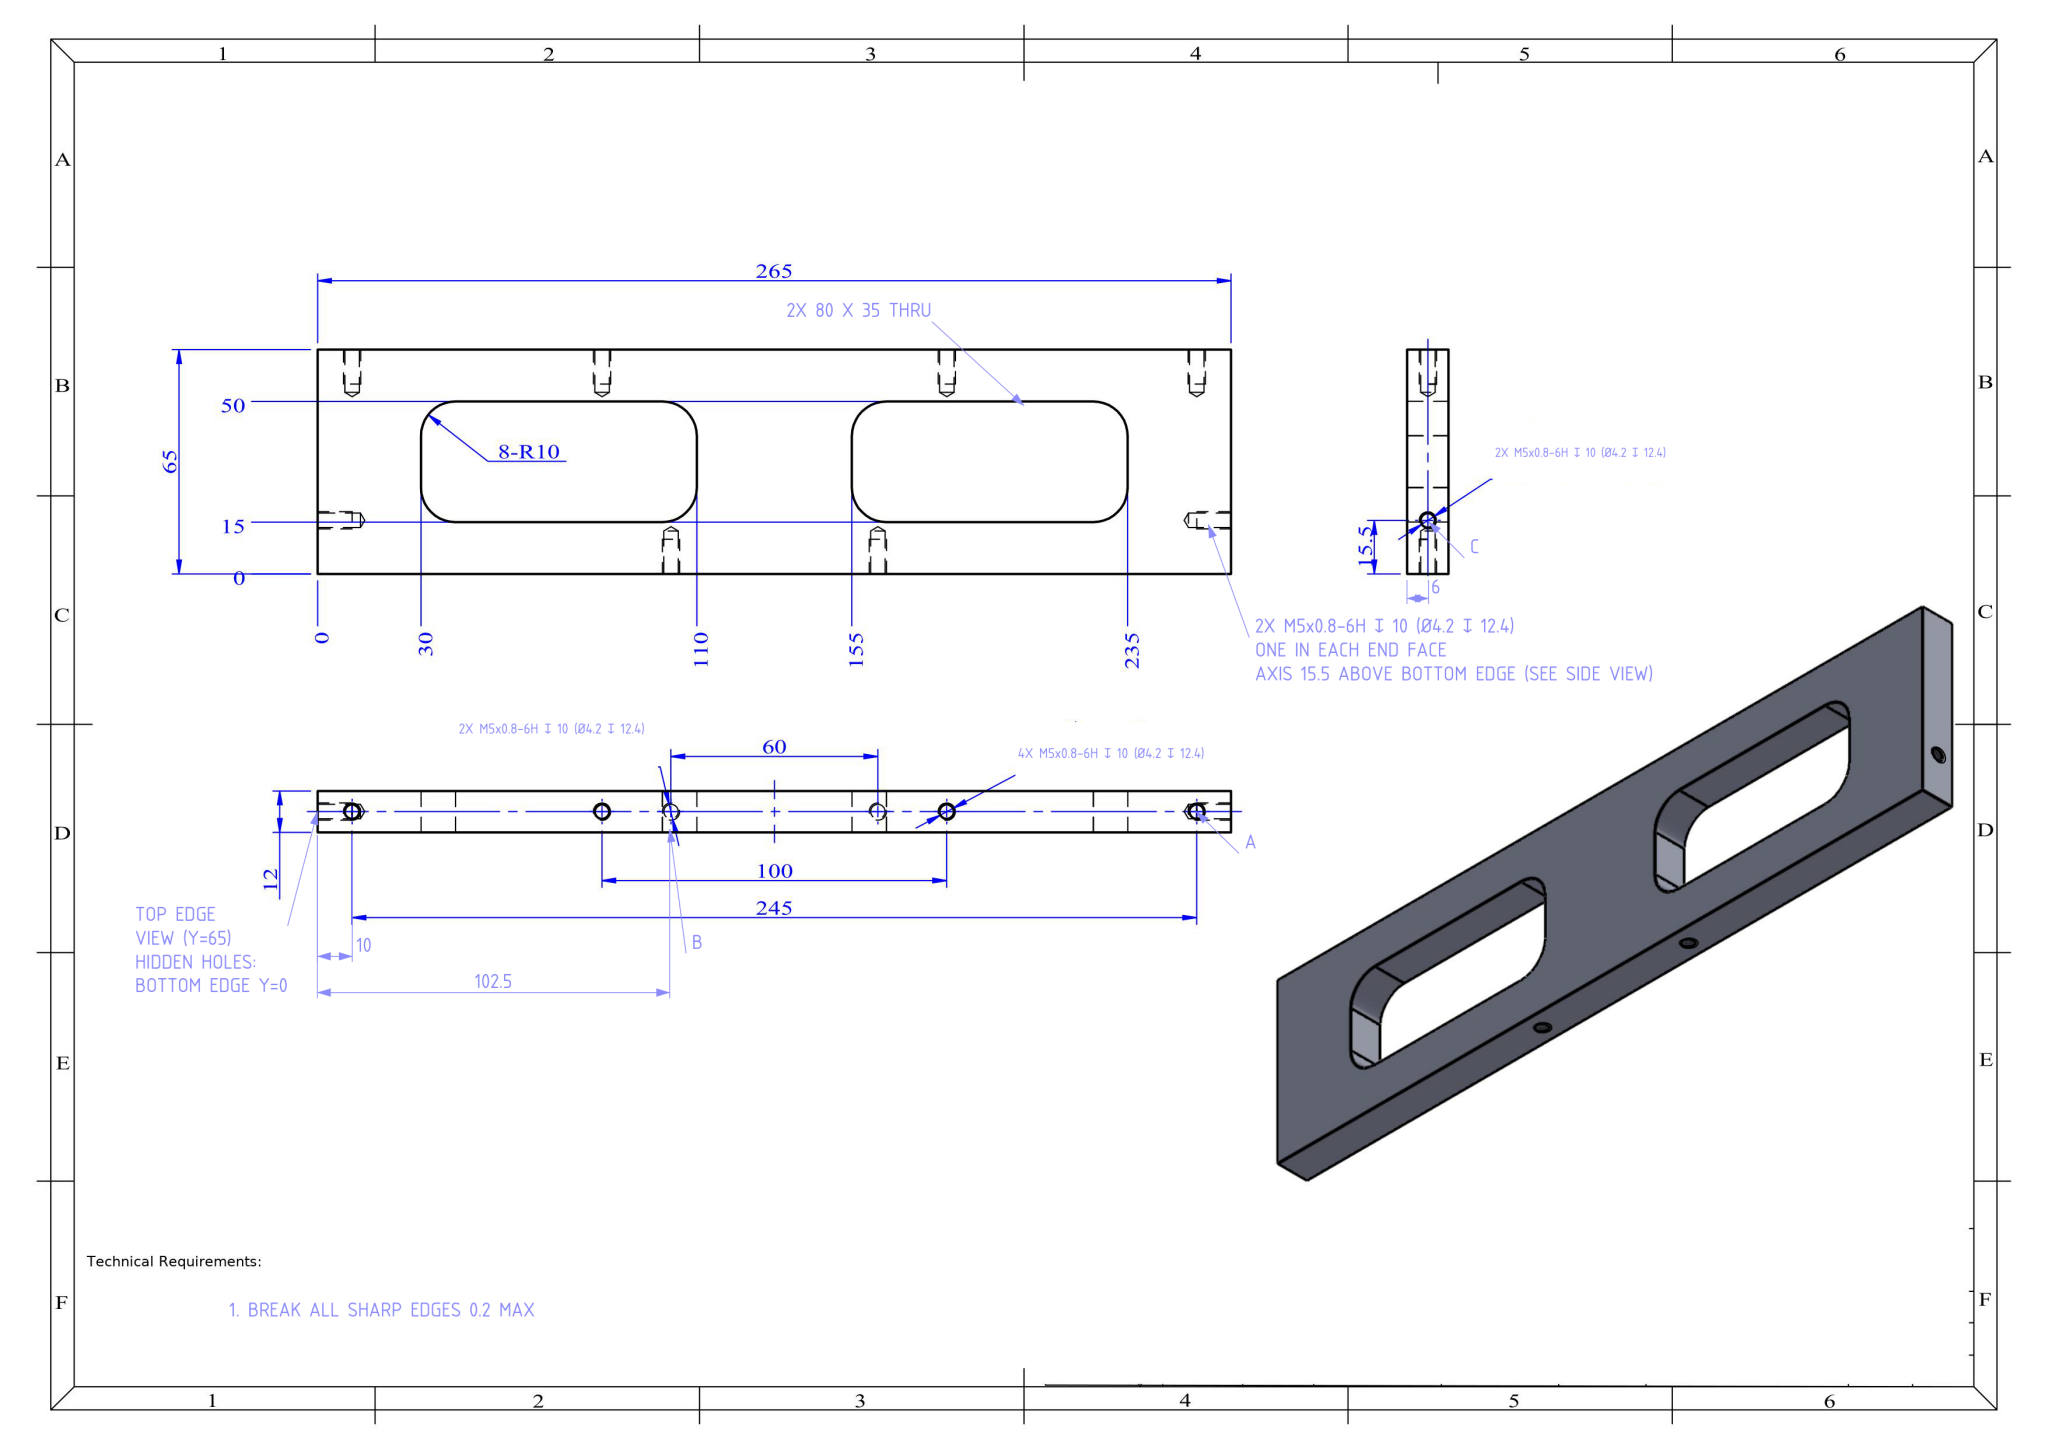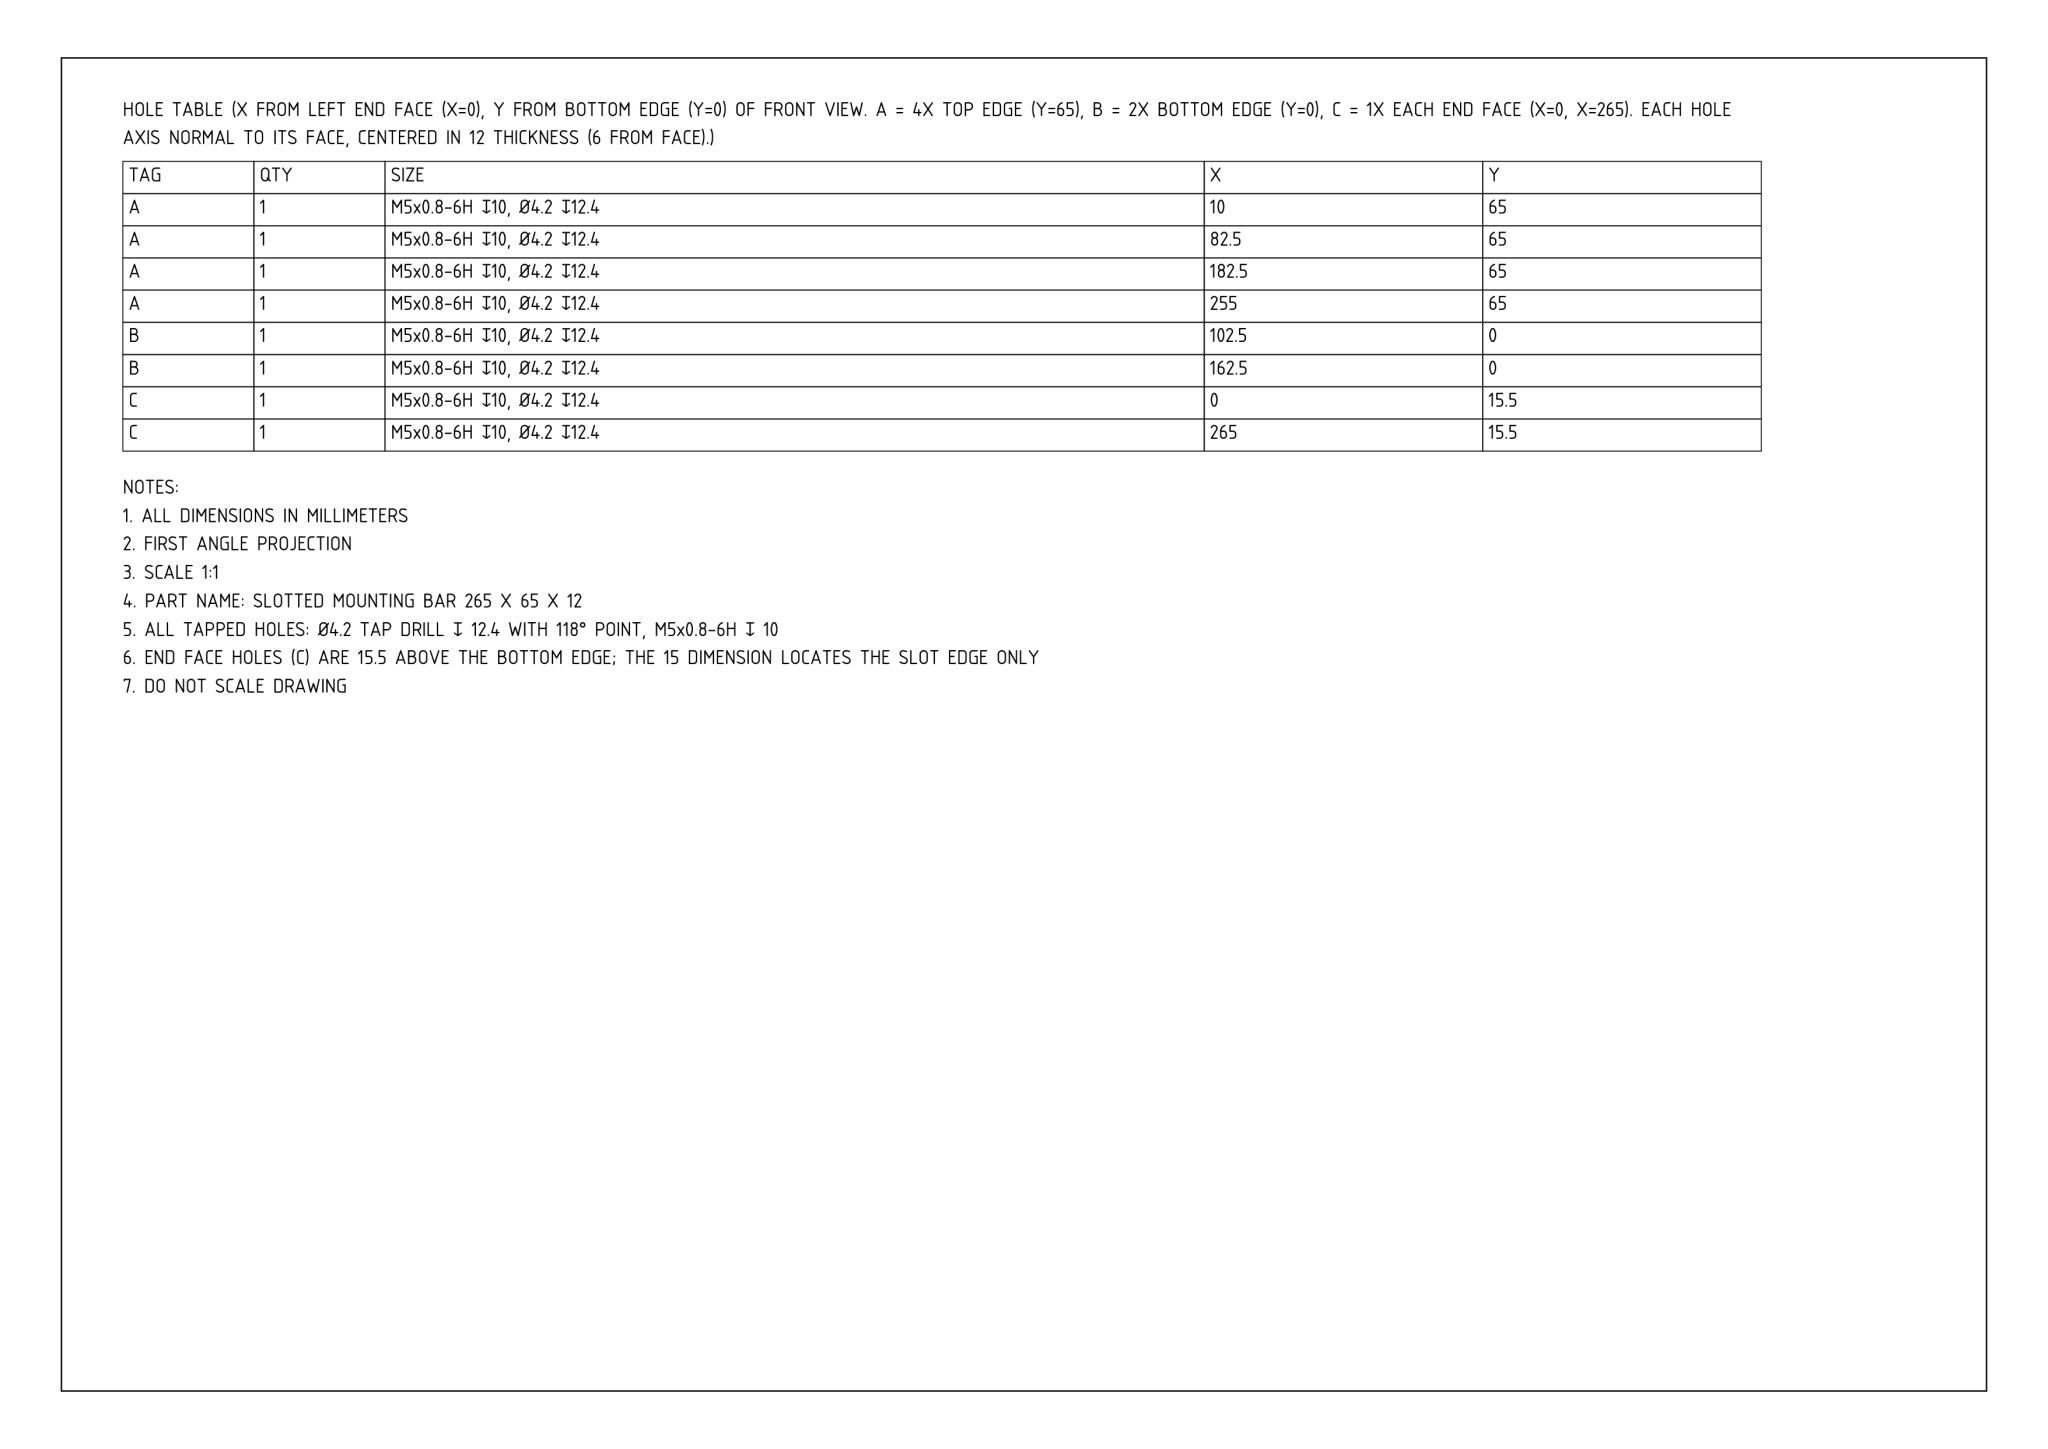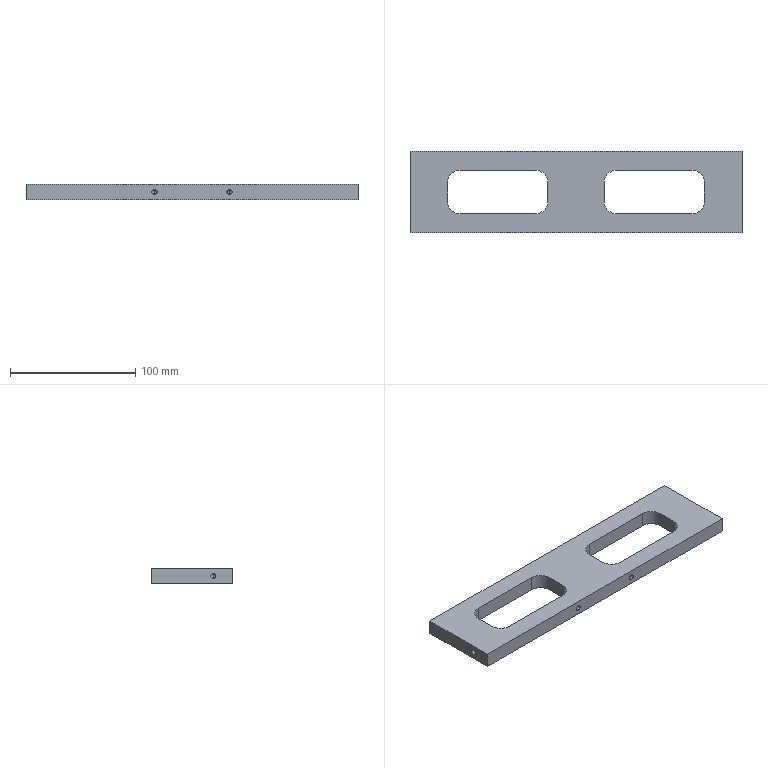Part | NX | mm | 1 solid | 54 faces | box 265 x 65 x 12 mm | volume 140139 mm3 | cylinder 24 | cone 16 | plane 14 | commonest cylinder face diameters 4.2 x16 20 x8